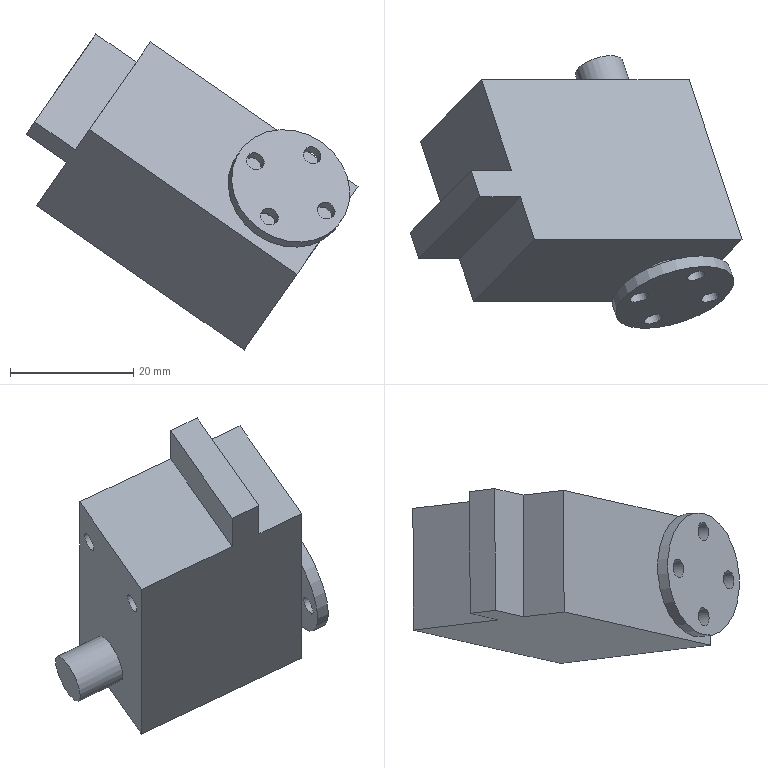Component | NX | SERVO | 2 solids | 25 faces | volume 26482 mm3 | plane 16 | cylinder 9 | commonest cylinder face diameters 3 x6 8 x2 20 x1